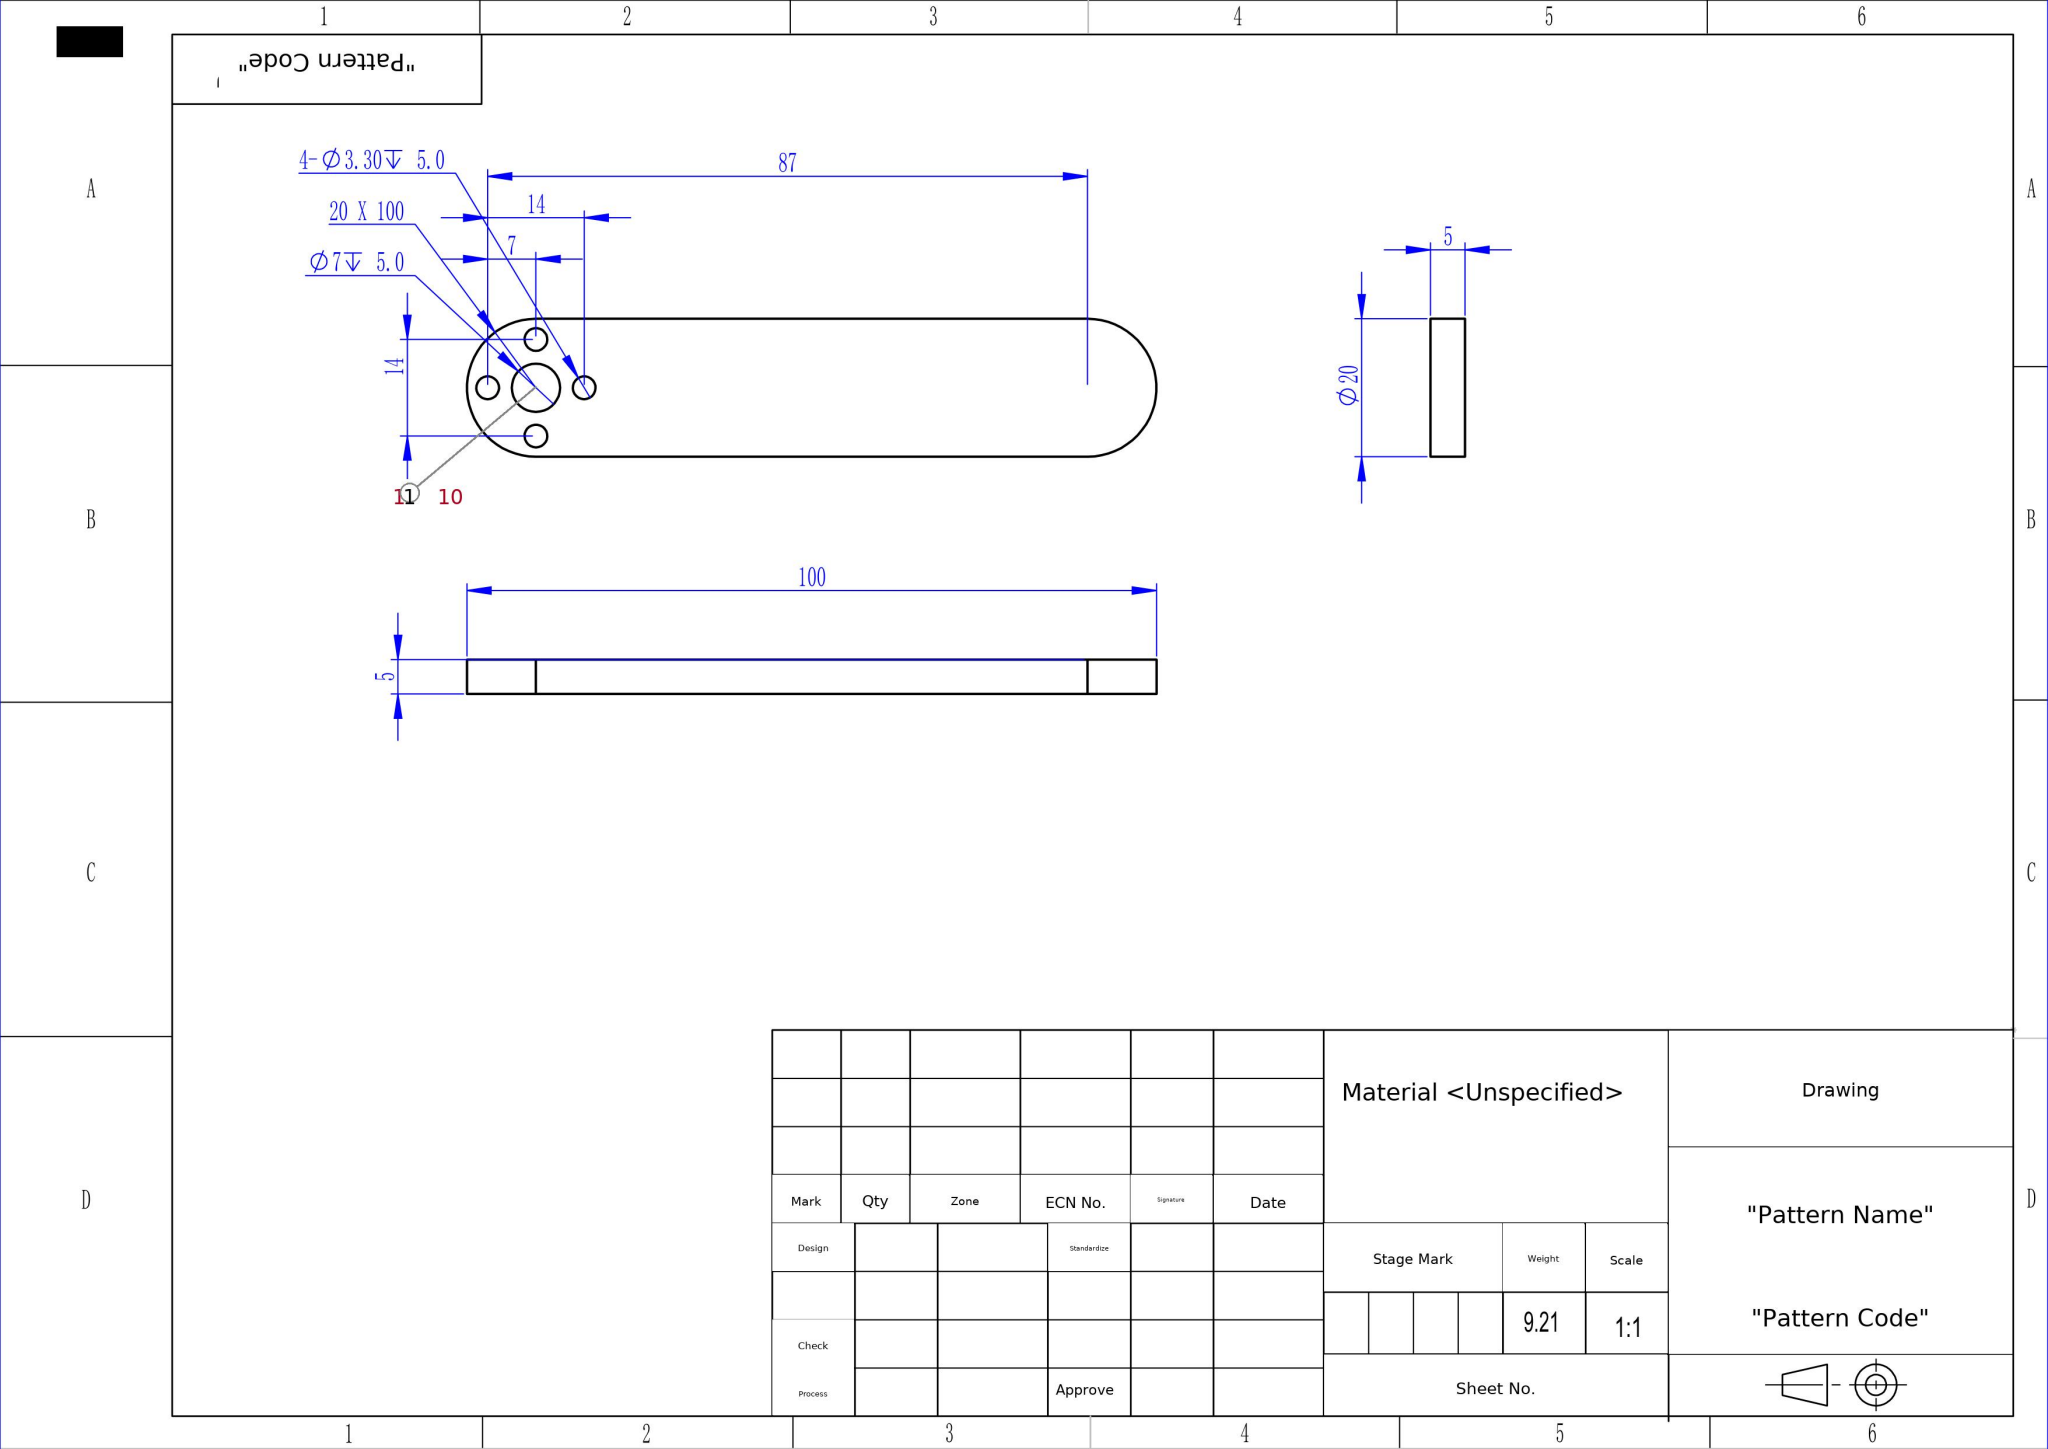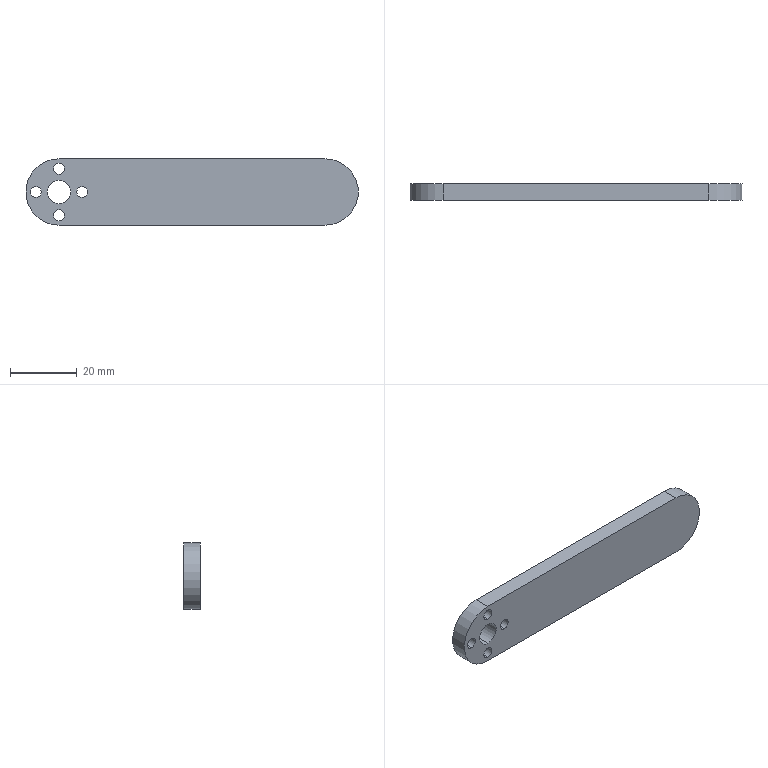Part | SolidWorks | mm | material <Unspecified> | 1 solid | 16 faces | box 100 x 5 x 20 mm | volume 9207 mm3 | cylinder 12 | plane 4 | commonest cylinder face diameters 3.3 x8 7 x2 20 x2
build123d program:
from build123d import *

# Parameters (mm, degrees)
BOSS_EXTRUDE1_DEPTH = 5
SKETCH2_R           = 1.65
SKETCH2_R_2         = 3.5
CUT_EXTRUDE1_DEPTH  = 5


with BuildPart() as part:
    # Sketch1 → Boss-Extrude1 (new body)
    with BuildSketch(Plane(origin=(0, 0, 0), x_dir=(1, 0, 0), z_dir=(0, 1, 0))):
        with BuildLine():
            Line((0, 10), (80, 10))
            ThreePointArc((80, 10), (90, 0), (80, -10))
            Line((80, -10), (0, -10))
            ThreePointArc((0, -10), (-10, 0), (0, 10))
        make_face()
    extrude(amount=BOSS_EXTRUDE1_DEPTH)

    # Sketch2 → Cut-Extrude1 (cut)
    with BuildSketch(Plane(origin=(0, 5, 0), x_dir=(1, 0, 0), z_dir=(0, 1, 0))):
        with Locations(Location((0, 7, 0), (0, 0, 270))):
            Circle(SKETCH2_R)
        with Locations(Location((-7, 0, 0), (0, 0, 270))):
            Circle(SKETCH2_R)
        with Locations(Location((0, -7, 0), (0, 0, 270))):
            Circle(SKETCH2_R)
        with Locations(Location((7, 0, 0), (0, 0, 270))):
            Circle(SKETCH2_R)
        with Locations(Location((0, 0, 0), (0, 0, 270))):
            Circle(SKETCH2_R_2)
    extrude(amount=-CUT_EXTRUDE1_DEPTH, mode=Mode.SUBTRACT)


solid = part.part
STEP:
#1=CARTESIAN_POINT('',(0.,0.,-8.65));
#2=VERTEX_POINT('',#1);
#3=CARTESIAN_POINT('',(0.,0.,-5.35));
#4=VERTEX_POINT('',#3);
#5=CARTESIAN_POINT('',(0.,0.,-7.));
#6=DIRECTION('',(0.,1.,0.));
#7=DIRECTION('',(0.,0.,1.));
#8=AXIS2_PLACEMENT_3D('',#5,#6,#7);
#9=CIRCLE('',#8,1.65);
#10=EDGE_CURVE('',#2,#4,#9,.T.);
#11=ORIENTED_EDGE('',*,*,#10,.F.);
#12=CARTESIAN_POINT('',(0.,5.,-8.65));
#13=VERTEX_POINT('',#12);
#14=CARTESIAN_POINT('',(0.,0.,-8.65));
#15=DIRECTION('',(0.,1.,0.));
#16=VECTOR('',#15,1000.);
#17=LINE('',#14,#16);
#18=EDGE_CURVE('',#2,#13,#17,.T.);
#19=ORIENTED_EDGE('',*,*,#18,.T.);
#20=CARTESIAN_POINT('',(0.,5.,-5.35));
#21=VERTEX_POINT('',#20);
#22=CARTESIAN_POINT('',(0.,5.,-7.));
#23=DIRECTION('',(0.,1.,0.));
#24=DIRECTION('',(0.,0.,1.));
#25=AXIS2_PLACEMENT_3D('',#22,#23,#24);
#26=CIRCLE('',#25,1.65);
#27=EDGE_CURVE('',#13,#21,#26,.T.);
#28=ORIENTED_EDGE('',*,*,#27,.T.);
#29=CARTESIAN_POINT('',(0.,0.,-5.35));
#30=DIRECTION('',(0.,1.,0.));
#31=VECTOR('',#30,1000.);
#32=LINE('',#29,#31);
#33=EDGE_CURVE('',#4,#21,#32,.T.);
#34=ORIENTED_EDGE('',*,*,#33,.F.);
#35=EDGE_LOOP('',(#11,#19,#28,#34));
#36=FACE_OUTER_BOUND('',#35,.T.);
#37=CARTESIAN_POINT('',(0.,0.,-7.));
#38=DIRECTION('',(0.,1.,0.));
#39=DIRECTION('',(0.,0.,1.));
#40=AXIS2_PLACEMENT_3D('',#37,#38,#39);
#41=CYLINDRICAL_SURFACE('',#40,1.65);
#42=ADVANCED_FACE('',(#36),#41,.F.);
#43=CARTESIAN_POINT('',(0.,0.,-3.5));
#44=VERTEX_POINT('',#43);
#45=CARTESIAN_POINT('',(0.,0.,3.5));
#46=VERTEX_POINT('',#45);
#47=CARTESIAN_POINT('',(0.,0.,0.));
#48=DIRECTION('',(0.,1.,0.));
#49=DIRECTION('',(0.,0.,1.));
#50=AXIS2_PLACEMENT_3D('',#47,#48,#49);
#51=CIRCLE('',#50,3.5);
#52=EDGE_CURVE('',#44,#46,#51,.T.);
#53=ORIENTED_EDGE('',*,*,#52,.F.);
#54=CARTESIAN_POINT('',(0.,5.,-3.5));
#55=VERTEX_POINT('',#54);
#56=CARTESIAN_POINT('',(0.,0.,-3.5));
#57=DIRECTION('',(0.,1.,0.));
#58=VECTOR('',#57,1000.);
#59=LINE('',#56,#58);
#60=EDGE_CURVE('',#44,#55,#59,.T.);
#61=ORIENTED_EDGE('',*,*,#60,.T.);
#62=CARTESIAN_POINT('',(0.,5.,3.5));
#63=VERTEX_POINT('',#62);
#64=CARTESIAN_POINT('',(0.,5.,0.));
#65=DIRECTION('',(0.,1.,0.));
#66=DIRECTION('',(0.,0.,1.));
#67=AXIS2_PLACEMENT_3D('',#64,#65,#66);
#68=CIRCLE('',#67,3.5);
#69=EDGE_CURVE('',#55,#63,#68,.T.);
#70=ORIENTED_EDGE('',*,*,#69,.T.);
#71=CARTESIAN_POINT('',(0.,0.,3.5));
#72=DIRECTION('',(0.,1.,0.));
#73=VECTOR('',#72,1000.);
#74=LINE('',#71,#73);
#75=EDGE_CURVE('',#46,#63,#74,.T.);
#76=ORIENTED_EDGE('',*,*,#75,.F.);
#77=EDGE_LOOP('',(#53,#61,#70,#76));
#78=FACE_OUTER_BOUND('',#77,.T.);
#79=CARTESIAN_POINT('',(0.,0.,0.));
#80=DIRECTION('',(0.,1.,0.));
#81=DIRECTION('',(0.,0.,1.));
#82=AXIS2_PLACEMENT_3D('',#79,#80,#81);
#83=CYLINDRICAL_SURFACE('',#82,3.5);
#84=ADVANCED_FACE('',(#78),#83,.F.);
#85=CARTESIAN_POINT('',(7.,0.,-1.65));
#86=VERTEX_POINT('',#85);
#87=CARTESIAN_POINT('',(7.,0.,1.65));
#88=VERTEX_POINT('',#87);
#89=CARTESIAN_POINT('',(7.,0.,0.));
#90=DIRECTION('',(0.,1.,0.));
#91=DIRECTION('',(0.,0.,1.));
#92=AXIS2_PLACEMENT_3D('',#89,#90,#91);
#93=CIRCLE('',#92,1.65);
#94=EDGE_CURVE('',#86,#88,#93,.T.);
#95=ORIENTED_EDGE('',*,*,#94,.F.);
#96=CARTESIAN_POINT('',(7.,5.,-1.65));
#97=VERTEX_POINT('',#96);
#98=CARTESIAN_POINT('',(7.,0.,-1.65));
#99=DIRECTION('',(0.,1.,0.));
#100=VECTOR('',#99,1000.);
#101=LINE('',#98,#100);
#102=EDGE_CURVE('',#86,#97,#101,.T.);
#103=ORIENTED_EDGE('',*,*,#102,.T.);
#104=CARTESIAN_POINT('',(7.,5.,1.65));
#105=VERTEX_POINT('',#104);
#106=CARTESIAN_POINT('',(7.,5.,0.));
#107=DIRECTION('',(0.,1.,0.));
#108=DIRECTION('',(0.,0.,1.));
#109=AXIS2_PLACEMENT_3D('',#106,#107,#108);
#110=CIRCLE('',#109,1.65);
#111=EDGE_CURVE('',#97,#105,#110,.T.);
#112=ORIENTED_EDGE('',*,*,#111,.T.);
#113=CARTESIAN_POINT('',(7.,0.,1.65));
#114=DIRECTION('',(0.,1.,0.));
#115=VECTOR('',#114,1000.);
#116=LINE('',#113,#115);
#117=EDGE_CURVE('',#88,#105,#116,.T.);
#118=ORIENTED_EDGE('',*,*,#117,.F.);
#119=EDGE_LOOP('',(#95,#103,#112,#118));
#120=FACE_OUTER_BOUND('',#119,.T.);
#121=CARTESIAN_POINT('',(7.,0.,0.));
#122=DIRECTION('',(0.,1.,0.));
#123=DIRECTION('',(0.,0.,1.));
#124=AXIS2_PLACEMENT_3D('',#121,#122,#123);
#125=CYLINDRICAL_SURFACE('',#124,1.65);
#126=ADVANCED_FACE('',(#120),#125,.F.);
#127=CARTESIAN_POINT('',(0.,0.,5.35));
#128=VERTEX_POINT('',#127);
#129=CARTESIAN_POINT('',(0.,0.,8.65));
#130=VERTEX_POINT('',#129);
#131=CARTESIAN_POINT('',(0.,0.,7.));
#132=DIRECTION('',(0.,1.,0.));
#133=DIRECTION('',(0.,0.,1.));
#134=AXIS2_PLACEMENT_3D('',#131,#132,#133);
#135=CIRCLE('',#134,1.65);
#136=EDGE_CURVE('',#128,#130,#135,.T.);
#137=ORIENTED_EDGE('',*,*,#136,.F.);
#138=CARTESIAN_POINT('',(0.,5.,5.35));
#139=VERTEX_POINT('',#138);
#140=CARTESIAN_POINT('',(0.,0.,5.35));
#141=DIRECTION('',(0.,1.,0.));
#142=VECTOR('',#141,1000.);
#143=LINE('',#140,#142);
#144=EDGE_CURVE('',#128,#139,#143,.T.);
#145=ORIENTED_EDGE('',*,*,#144,.T.);
#146=CARTESIAN_POINT('',(0.,5.,8.65));
#147=VERTEX_POINT('',#146);
#148=CARTESIAN_POINT('',(0.,5.,7.));
#149=DIRECTION('',(0.,1.,0.));
#150=DIRECTION('',(0.,0.,1.));
#151=AXIS2_PLACEMENT_3D('',#148,#149,#150);
#152=CIRCLE('',#151,1.65);
#153=EDGE_CURVE('',#139,#147,#152,.T.);
#154=ORIENTED_EDGE('',*,*,#153,.T.);
#155=CARTESIAN_POINT('',(0.,0.,8.65));
#156=DIRECTION('',(0.,1.,0.));
#157=VECTOR('',#156,1000.);
#158=LINE('',#155,#157);
#159=EDGE_CURVE('',#130,#147,#158,.T.);
#160=ORIENTED_EDGE('',*,*,#159,.F.);
#161=EDGE_LOOP('',(#137,#145,#154,#160));
#162=FACE_OUTER_BOUND('',#161,.T.);
#163=CARTESIAN_POINT('',(0.,0.,7.));
#164=DIRECTION('',(0.,1.,0.));
#165=DIRECTION('',(0.,0.,1.));
#166=AXIS2_PLACEMENT_3D('',#163,#164,#165);
#167=CYLINDRICAL_SURFACE('',#166,1.65);
#168=ADVANCED_FACE('',(#162),#167,.F.);
#169=CARTESIAN_POINT('',(-7.,0.,-1.65));
#170=VERTEX_POINT('',#169);
#171=CARTESIAN_POINT('',(-7.,0.,1.65));
#172=VERTEX_POINT('',#171);
#173=CARTESIAN_POINT('',(-7.,0.,0.));
#174=DIRECTION('',(0.,1.,0.));
#175=DIRECTION('',(0.,0.,1.));
#176=AXIS2_PLACEMENT_3D('',#173,#174,#175);
#177=CIRCLE('',#176,1.65);
#178=EDGE_CURVE('',#170,#172,#177,.T.);
#179=ORIENTED_EDGE('',*,*,#178,.F.);
#180=CARTESIAN_POINT('',(-7.,5.,-1.65));
#181=VERTEX_POINT('',#180);
#182=CARTESIAN_POINT('',(-7.,0.,-1.65));
#183=DIRECTION('',(0.,1.,0.));
#184=VECTOR('',#183,1000.);
#185=LINE('',#182,#184);
#186=EDGE_CURVE('',#170,#181,#185,.T.);
#187=ORIENTED_EDGE('',*,*,#186,.T.);
#188=CARTESIAN_POINT('',(-7.,5.,1.65));
#189=VERTEX_POINT('',#188);
#190=CARTESIAN_POINT('',(-7.,5.,0.));
#191=DIRECTION('',(0.,1.,0.));
#192=DIRECTION('',(0.,0.,1.));
#193=AXIS2_PLACEMENT_3D('',#190,#191,#192);
#194=CIRCLE('',#193,1.65);
#195=EDGE_CURVE('',#181,#189,#194,.T.);
#196=ORIENTED_EDGE('',*,*,#195,.T.);
#197=CARTESIAN_POINT('',(-7.,0.,1.65));
#198=DIRECTION('',(0.,1.,0.));
#199=VECTOR('',#198,1000.);
#200=LINE('',#197,#199);
#201=EDGE_CURVE('',#172,#189,#200,.T.);
#202=ORIENTED_EDGE('',*,*,#201,.F.);
#203=EDGE_LOOP('',(#179,#187,#196,#202));
#204=FACE_OUTER_BOUND('',#203,.T.);
#205=CARTESIAN_POINT('',(-7.,0.,0.));
#206=DIRECTION('',(0.,1.,0.));
#207=DIRECTION('',(0.,0.,1.));
#208=AXIS2_PLACEMENT_3D('',#205,#206,#207);
#209=CYLINDRICAL_SURFACE('',#208,1.65);
#210=ADVANCED_FACE('',(#204),#209,.F.);
#211=CARTESIAN_POINT('',(0.,0.,-10.));
#212=VERTEX_POINT('',#211);
#213=CARTESIAN_POINT('',(0.,0.,10.));
#214=VERTEX_POINT('',#213);
#215=CARTESIAN_POINT('',(0.,0.,0.));
#216=DIRECTION('',(0.,1.,0.));
#217=DIRECTION('',(0.,0.,1.));
#218=AXIS2_PLACEMENT_3D('',#215,#216,#217);
#219=CIRCLE('',#218,10.);
#220=EDGE_CURVE('',#212,#214,#219,.T.);
#221=ORIENTED_EDGE('',*,*,#220,.T.);
#222=CARTESIAN_POINT('',(0.,5.,10.));
#223=VERTEX_POINT('',#222);
#224=CARTESIAN_POINT('',(0.,5.,10.));
#225=DIRECTION('',(0.,-1.,0.));
#226=VECTOR('',#225,1000.);
#227=LINE('',#224,#226);
#228=EDGE_CURVE('',#223,#214,#227,.T.);
#229=ORIENTED_EDGE('',*,*,#228,.F.);
#230=CARTESIAN_POINT('',(0.,5.,-10.));
#231=VERTEX_POINT('',#230);
#232=CARTESIAN_POINT('',(0.,5.,0.));
#233=DIRECTION('',(0.,1.,0.));
#234=DIRECTION('',(0.,0.,1.));
#235=AXIS2_PLACEMENT_3D('',#232,#233,#234);
#236=CIRCLE('',#235,10.);
#237=EDGE_CURVE('',#231,#223,#236,.T.);
#238=ORIENTED_EDGE('',*,*,#237,.F.);
#239=CARTESIAN_POINT('',(0.,5.,-10.));
#240=DIRECTION('',(0.,-1.,0.));
#241=VECTOR('',#240,1000.);
#242=LINE('',#239,#241);
#243=EDGE_CURVE('',#231,#212,#242,.T.);
#244=ORIENTED_EDGE('',*,*,#243,.T.);
#245=EDGE_LOOP('',(#221,#229,#238,#244));
#246=FACE_OUTER_BOUND('',#245,.T.);
#247=CARTESIAN_POINT('',(0.,5.,0.));
#248=DIRECTION('',(0.,-1.,0.));
#249=DIRECTION('',(0.,0.,-1.));
#250=AXIS2_PLACEMENT_3D('',#247,#248,#249);
#251=CYLINDRICAL_SURFACE('',#250,10.);
#252=ADVANCED_FACE('',(#246),#251,.T.);
#253=CARTESIAN_POINT('',(80.,0.,10.));
#254=VERTEX_POINT('',#253);
#255=CARTESIAN_POINT('',(0.,0.,10.));
#256=DIRECTION('',(1.,0.,0.));
#257=VECTOR('',#256,1000.);
#258=LINE('',#255,#257);
#259=EDGE_CURVE('',#214,#254,#258,.T.);
#260=ORIENTED_EDGE('',*,*,#259,.T.);
#261=CARTESIAN_POINT('',(80.,5.,10.));
#262=VERTEX_POINT('',#261);
#263=CARTESIAN_POINT('',(80.,5.,10.));
#264=DIRECTION('',(0.,-1.,0.));
#265=VECTOR('',#264,1000.);
#266=LINE('',#263,#265);
#267=EDGE_CURVE('',#262,#254,#266,.T.);
#268=ORIENTED_EDGE('',*,*,#267,.F.);
#269=CARTESIAN_POINT('',(0.,5.,10.));
#270=DIRECTION('',(1.,0.,0.));
#271=VECTOR('',#270,1000.);
#272=LINE('',#269,#271);
#273=EDGE_CURVE('',#223,#262,#272,.T.);
#274=ORIENTED_EDGE('',*,*,#273,.F.);
#275=ORIENTED_EDGE('',*,*,#228,.T.);
#276=EDGE_LOOP('',(#260,#268,#274,#275));
#277=FACE_OUTER_BOUND('',#276,.T.);
#278=CARTESIAN_POINT('',(0.,5.,10.));
#279=DIRECTION('',(0.,0.,-1.));
#280=DIRECTION('',(-1.,0.,0.));
#281=AXIS2_PLACEMENT_3D('',#278,#279,#280);
#282=PLANE('',#281);
#283=ADVANCED_FACE('',(#277),#282,.F.);
#284=CARTESIAN_POINT('',(80.,0.,-10.));
#285=VERTEX_POINT('',#284);
#286=CARTESIAN_POINT('',(80.,0.,0.));
#287=DIRECTION('',(0.,1.,0.));
#288=DIRECTION('',(0.,0.,1.));
#289=AXIS2_PLACEMENT_3D('',#286,#287,#288);
#290=CIRCLE('',#289,10.);
#291=EDGE_CURVE('',#254,#285,#290,.T.);
#292=ORIENTED_EDGE('',*,*,#291,.T.);
#293=CARTESIAN_POINT('',(80.,5.,-10.));
#294=VERTEX_POINT('',#293);
#295=CARTESIAN_POINT('',(80.,5.,-10.));
#296=DIRECTION('',(0.,-1.,0.));
#297=VECTOR('',#296,1000.);
#298=LINE('',#295,#297);
#299=EDGE_CURVE('',#294,#285,#298,.T.);
#300=ORIENTED_EDGE('',*,*,#299,.F.);
#301=CARTESIAN_POINT('',(80.,5.,0.));
#302=DIRECTION('',(0.,1.,0.));
#303=DIRECTION('',(0.,0.,1.));
#304=AXIS2_PLACEMENT_3D('',#301,#302,#303);
#305=CIRCLE('',#304,10.);
#306=EDGE_CURVE('',#262,#294,#305,.T.);
#307=ORIENTED_EDGE('',*,*,#306,.F.);
#308=ORIENTED_EDGE('',*,*,#267,.T.);
#309=EDGE_LOOP('',(#292,#300,#307,#308));
#310=FACE_OUTER_BOUND('',#309,.T.);
#311=CARTESIAN_POINT('',(80.,5.,0.));
#312=DIRECTION('',(0.,-1.,0.));
#313=DIRECTION('',(0.,0.,-1.));
#314=AXIS2_PLACEMENT_3D('',#311,#312,#313);
#315=CYLINDRICAL_SURFACE('',#314,10.);
#316=ADVANCED_FACE('',(#310),#315,.T.);
#317=CARTESIAN_POINT('',(0.,0.,-10.));
#318=DIRECTION('',(-1.,0.,0.));
#319=VECTOR('',#318,1000.);
#320=LINE('',#317,#319);
#321=EDGE_CURVE('',#285,#212,#320,.T.);
#322=ORIENTED_EDGE('',*,*,#321,.T.);
#323=ORIENTED_EDGE('',*,*,#243,.F.);
#324=CARTESIAN_POINT('',(0.,5.,-10.));
#325=DIRECTION('',(-1.,0.,0.));
#326=VECTOR('',#325,1000.);
#327=LINE('',#324,#326);
#328=EDGE_CURVE('',#294,#231,#327,.T.);
#329=ORIENTED_EDGE('',*,*,#328,.F.);
#330=ORIENTED_EDGE('',*,*,#299,.T.);
#331=EDGE_LOOP('',(#322,#323,#329,#330));
#332=FACE_OUTER_BOUND('',#331,.T.);
#333=CARTESIAN_POINT('',(0.,5.,-10.));
#334=DIRECTION('',(0.,0.,1.));
#335=DIRECTION('',(1.,0.,0.));
#336=AXIS2_PLACEMENT_3D('',#333,#334,#335);
#337=PLANE('',#336);
#338=ADVANCED_FACE('',(#332),#337,.F.);
#339=CARTESIAN_POINT('',(0.,5.,-7.));
#340=DIRECTION('',(0.,1.,0.));
#341=DIRECTION('',(0.,0.,1.));
#342=AXIS2_PLACEMENT_3D('',#339,#340,#341);
#343=CIRCLE('',#342,1.65);
#344=EDGE_CURVE('',#21,#13,#343,.T.);
#345=ORIENTED_EDGE('',*,*,#344,.F.);
#346=ORIENTED_EDGE('',*,*,#27,.F.);
#347=EDGE_LOOP('',(#345,#346));
#348=FACE_BOUND('',#347,.T.);
#349=CARTESIAN_POINT('',(0.,5.,0.));
#350=DIRECTION('',(0.,1.,0.));
#351=DIRECTION('',(0.,0.,1.));
#352=AXIS2_PLACEMENT_3D('',#349,#350,#351);
#353=CIRCLE('',#352,3.5);
#354=EDGE_CURVE('',#63,#55,#353,.T.);
#355=ORIENTED_EDGE('',*,*,#354,.F.);
#356=ORIENTED_EDGE('',*,*,#69,.F.);
#357=EDGE_LOOP('',(#355,#356));
#358=FACE_BOUND('',#357,.T.);
#359=CARTESIAN_POINT('',(7.,5.,0.));
#360=DIRECTION('',(0.,1.,0.));
#361=DIRECTION('',(0.,0.,1.));
#362=AXIS2_PLACEMENT_3D('',#359,#360,#361);
#363=CIRCLE('',#362,1.65);
#364=EDGE_CURVE('',#105,#97,#363,.T.);
#365=ORIENTED_EDGE('',*,*,#364,.F.);
#366=ORIENTED_EDGE('',*,*,#111,.F.);
#367=EDGE_LOOP('',(#365,#366));
#368=FACE_BOUND('',#367,.T.);
#369=CARTESIAN_POINT('',(0.,5.,7.));
#370=DIRECTION('',(0.,1.,0.));
#371=DIRECTION('',(0.,0.,1.));
#372=AXIS2_PLACEMENT_3D('',#369,#370,#371);
#373=CIRCLE('',#372,1.65);
#374=EDGE_CURVE('',#147,#139,#373,.T.);
#375=ORIENTED_EDGE('',*,*,#374,.F.);
#376=ORIENTED_EDGE('',*,*,#153,.F.);
#377=EDGE_LOOP('',(#375,#376));
#378=FACE_BOUND('',#377,.T.);
#379=CARTESIAN_POINT('',(-7.,5.,0.));
#380=DIRECTION('',(0.,1.,0.));
#381=DIRECTION('',(0.,0.,1.));
#382=AXIS2_PLACEMENT_3D('',#379,#380,#381);
#383=CIRCLE('',#382,1.65);
#384=EDGE_CURVE('',#189,#181,#383,.T.);
#385=ORIENTED_EDGE('',*,*,#384,.F.);
#386=ORIENTED_EDGE('',*,*,#195,.F.);
#387=EDGE_LOOP('',(#385,#386));
#388=FACE_BOUND('',#387,.T.);
#389=ORIENTED_EDGE('',*,*,#237,.T.);
#390=ORIENTED_EDGE('',*,*,#273,.T.);
#391=ORIENTED_EDGE('',*,*,#306,.T.);
#392=ORIENTED_EDGE('',*,*,#328,.T.);
#393=EDGE_LOOP('',(#389,#390,#391,#392));
#394=FACE_OUTER_BOUND('',#393,.T.);
#395=CARTESIAN_POINT('',(0.,5.,0.));
#396=DIRECTION('',(0.,1.,0.));
#397=DIRECTION('',(0.,0.,1.));
#398=AXIS2_PLACEMENT_3D('',#395,#396,#397);
#399=PLANE('',#398);
#400=ADVANCED_FACE('',(#348,#358,#368,#378,#388,#394),#399,.T.);
#401=CARTESIAN_POINT('',(0.,0.,-7.));
#402=DIRECTION('',(0.,1.,0.));
#403=DIRECTION('',(0.,0.,1.));
#404=AXIS2_PLACEMENT_3D('',#401,#402,#403);
#405=CIRCLE('',#404,1.65);
#406=EDGE_CURVE('',#4,#2,#405,.T.);
#407=ORIENTED_EDGE('',*,*,#406,.T.);
#408=ORIENTED_EDGE('',*,*,#10,.T.);
#409=EDGE_LOOP('',(#407,#408));
#410=FACE_BOUND('',#409,.T.);
#411=CARTESIAN_POINT('',(0.,0.,0.));
#412=DIRECTION('',(0.,1.,0.));
#413=DIRECTION('',(0.,0.,1.));
#414=AXIS2_PLACEMENT_3D('',#411,#412,#413);
#415=CIRCLE('',#414,3.5);
#416=EDGE_CURVE('',#46,#44,#415,.T.);
#417=ORIENTED_EDGE('',*,*,#416,.T.);
#418=ORIENTED_EDGE('',*,*,#52,.T.);
#419=EDGE_LOOP('',(#417,#418));
#420=FACE_BOUND('',#419,.T.);
#421=CARTESIAN_POINT('',(7.,0.,0.));
#422=DIRECTION('',(0.,1.,0.));
#423=DIRECTION('',(0.,0.,1.));
#424=AXIS2_PLACEMENT_3D('',#421,#422,#423);
#425=CIRCLE('',#424,1.65);
#426=EDGE_CURVE('',#88,#86,#425,.T.);
#427=ORIENTED_EDGE('',*,*,#426,.T.);
#428=ORIENTED_EDGE('',*,*,#94,.T.);
#429=EDGE_LOOP('',(#427,#428));
#430=FACE_BOUND('',#429,.T.);
#431=CARTESIAN_POINT('',(0.,0.,7.));
#432=DIRECTION('',(0.,1.,0.));
#433=DIRECTION('',(0.,0.,1.));
#434=AXIS2_PLACEMENT_3D('',#431,#432,#433);
#435=CIRCLE('',#434,1.65);
#436=EDGE_CURVE('',#130,#128,#435,.T.);
#437=ORIENTED_EDGE('',*,*,#436,.T.);
#438=ORIENTED_EDGE('',*,*,#136,.T.);
#439=EDGE_LOOP('',(#437,#438));
#440=FACE_BOUND('',#439,.T.);
#441=CARTESIAN_POINT('',(-7.,0.,0.));
#442=DIRECTION('',(0.,1.,0.));
#443=DIRECTION('',(0.,0.,1.));
#444=AXIS2_PLACEMENT_3D('',#441,#442,#443);
#445=CIRCLE('',#444,1.65);
#446=EDGE_CURVE('',#172,#170,#445,.T.);
#447=ORIENTED_EDGE('',*,*,#446,.T.);
#448=ORIENTED_EDGE('',*,*,#178,.T.);
#449=EDGE_LOOP('',(#447,#448));
#450=FACE_BOUND('',#449,.T.);
#451=ORIENTED_EDGE('',*,*,#220,.F.);
#452=ORIENTED_EDGE('',*,*,#321,.F.);
#453=ORIENTED_EDGE('',*,*,#291,.F.);
#454=ORIENTED_EDGE('',*,*,#259,.F.);
#455=EDGE_LOOP('',(#451,#452,#453,#454));
#456=FACE_OUTER_BOUND('',#455,.T.);
#457=CARTESIAN_POINT('',(0.,0.,0.));
#458=DIRECTION('',(0.,1.,0.));
#459=DIRECTION('',(0.,0.,1.));
#460=AXIS2_PLACEMENT_3D('',#457,#458,#459);
#461=PLANE('',#460);
#462=ADVANCED_FACE('',(#410,#420,#430,#440,#450,#456),#461,.F.);
#463=ORIENTED_EDGE('',*,*,#186,.F.);
#464=ORIENTED_EDGE('',*,*,#446,.F.);
#465=ORIENTED_EDGE('',*,*,#201,.T.);
#466=ORIENTED_EDGE('',*,*,#384,.T.);
#467=EDGE_LOOP('',(#463,#464,#465,#466));
#468=FACE_OUTER_BOUND('',#467,.T.);
#469=CARTESIAN_POINT('',(-7.,0.,0.));
#470=DIRECTION('',(0.,1.,0.));
#471=DIRECTION('',(0.,0.,1.));
#472=AXIS2_PLACEMENT_3D('',#469,#470,#471);
#473=CYLINDRICAL_SURFACE('',#472,1.65);
#474=ADVANCED_FACE('',(#468),#473,.F.);
#475=ORIENTED_EDGE('',*,*,#144,.F.);
#476=ORIENTED_EDGE('',*,*,#436,.F.);
#477=ORIENTED_EDGE('',*,*,#159,.T.);
#478=ORIENTED_EDGE('',*,*,#374,.T.);
#479=EDGE_LOOP('',(#475,#476,#477,#478));
#480=FACE_OUTER_BOUND('',#479,.T.);
#481=CARTESIAN_POINT('',(0.,0.,7.));
#482=DIRECTION('',(0.,1.,0.));
#483=DIRECTION('',(0.,0.,1.));
#484=AXIS2_PLACEMENT_3D('',#481,#482,#483);
#485=CYLINDRICAL_SURFACE('',#484,1.65);
#486=ADVANCED_FACE('',(#480),#485,.F.);
#487=ORIENTED_EDGE('',*,*,#102,.F.);
#488=ORIENTED_EDGE('',*,*,#426,.F.);
#489=ORIENTED_EDGE('',*,*,#117,.T.);
#490=ORIENTED_EDGE('',*,*,#364,.T.);
#491=EDGE_LOOP('',(#487,#488,#489,#490));
#492=FACE_OUTER_BOUND('',#491,.T.);
#493=CARTESIAN_POINT('',(7.,0.,0.));
#494=DIRECTION('',(0.,1.,0.));
#495=DIRECTION('',(0.,0.,1.));
#496=AXIS2_PLACEMENT_3D('',#493,#494,#495);
#497=CYLINDRICAL_SURFACE('',#496,1.65);
#498=ADVANCED_FACE('',(#492),#497,.F.);
#499=ORIENTED_EDGE('',*,*,#60,.F.);
#500=ORIENTED_EDGE('',*,*,#416,.F.);
#501=ORIENTED_EDGE('',*,*,#75,.T.);
#502=ORIENTED_EDGE('',*,*,#354,.T.);
#503=EDGE_LOOP('',(#499,#500,#501,#502));
#504=FACE_OUTER_BOUND('',#503,.T.);
#505=CARTESIAN_POINT('',(0.,0.,0.));
#506=DIRECTION('',(0.,1.,0.));
#507=DIRECTION('',(0.,0.,1.));
#508=AXIS2_PLACEMENT_3D('',#505,#506,#507);
#509=CYLINDRICAL_SURFACE('',#508,3.5);
#510=ADVANCED_FACE('',(#504),#509,.F.);
#511=ORIENTED_EDGE('',*,*,#18,.F.);
#512=ORIENTED_EDGE('',*,*,#406,.F.);
#513=ORIENTED_EDGE('',*,*,#33,.T.);
#514=ORIENTED_EDGE('',*,*,#344,.T.);
#515=EDGE_LOOP('',(#511,#512,#513,#514));
#516=FACE_OUTER_BOUND('',#515,.T.);
#517=CARTESIAN_POINT('',(0.,0.,-7.));
#518=DIRECTION('',(0.,1.,0.));
#519=DIRECTION('',(0.,0.,1.));
#520=AXIS2_PLACEMENT_3D('',#517,#518,#519);
#521=CYLINDRICAL_SURFACE('',#520,1.65);
#522=ADVANCED_FACE('',(#516),#521,.F.);
#523=CLOSED_SHELL('',(#42,#84,#126,#168,#210,#252,#283,#316,#338,#400,#462,#474,#486,#498,#510,#522));
#524=MANIFOLD_SOLID_BREP('',#523);
#525=CARTESIAN_POINT('',(0.,0.,0.));
#526=DIRECTION('',(0.,0.,1.));
#527=DIRECTION('',(1.,0.,0.));
#528=AXIS2_PLACEMENT_3D('',#525,#526,#527);
#529=(LENGTH_UNIT()NAMED_UNIT(*)SI_UNIT(.MILLI.,.METRE.));
#530=UNCERTAINTY_MEASURE_WITH_UNIT(LENGTH_MEASURE(0.00001),#529,'','');
#531=(NAMED_UNIT(*)PLANE_ANGLE_UNIT()SI_UNIT($,.RADIAN.));
#532=(NAMED_UNIT(*)SI_UNIT($,.STERADIAN.)SOLID_ANGLE_UNIT());
#533=(GEOMETRIC_REPRESENTATION_CONTEXT(3)GLOBAL_UNCERTAINTY_ASSIGNED_CONTEXT((#530))GLOBAL_UNIT_ASSIGNED_CONTEXT((#529,#531,#532))REPRESENTATION_CONTEXT('',''));
#534=ADVANCED_BREP_SHAPE_REPRESENTATION('',(#524,#528),#533);